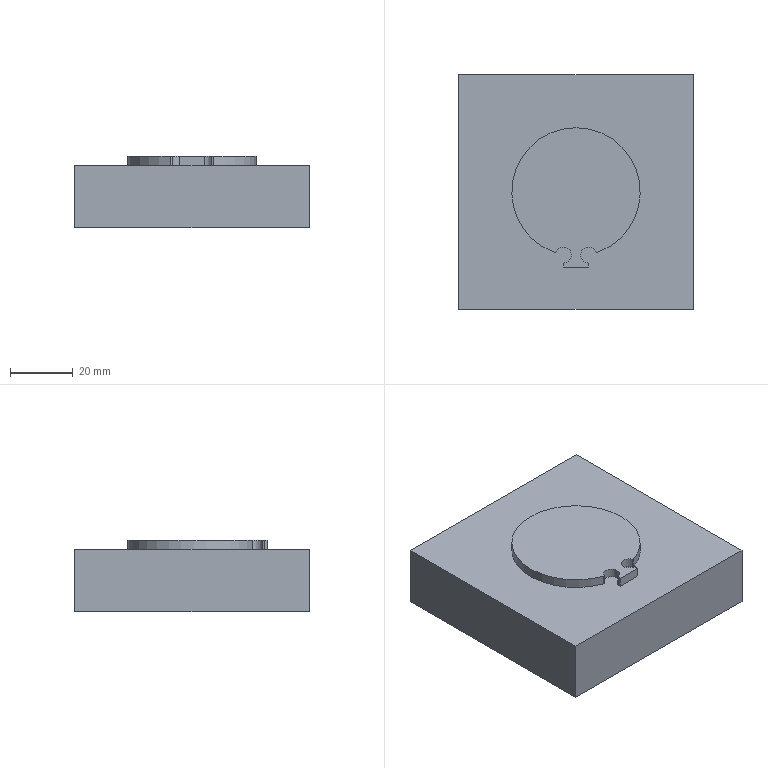CAM job | Mastercam | mm | 7 operations | part box 75 x 75 x 23
1. Facing | 24 - 100 平铣刀
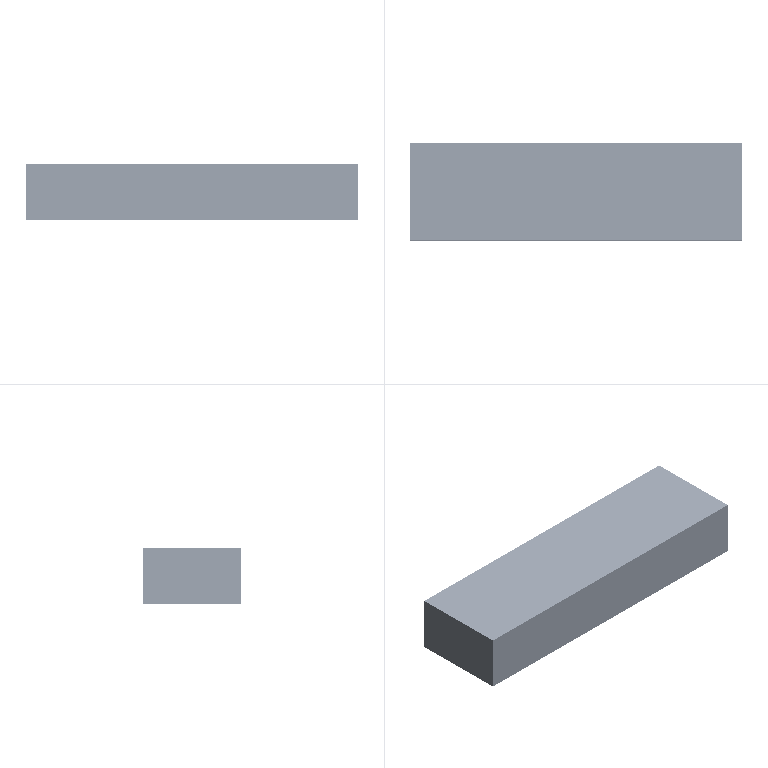2. 2D High Speed (2D Area Mill) | 10 - 10 平铣刀
3. Contour (Remachining) | 4 - 4 平铣刀
4. 2D High Speed (2D Area Mill) | 4 - 4 平铣刀
5. Contour (2D) | 4 - 4 平铣刀
6. Contour (2D chamfer) | 7 - 4 倒角刀
7. Drill/Counterbore | 7 - 4 倒角刀